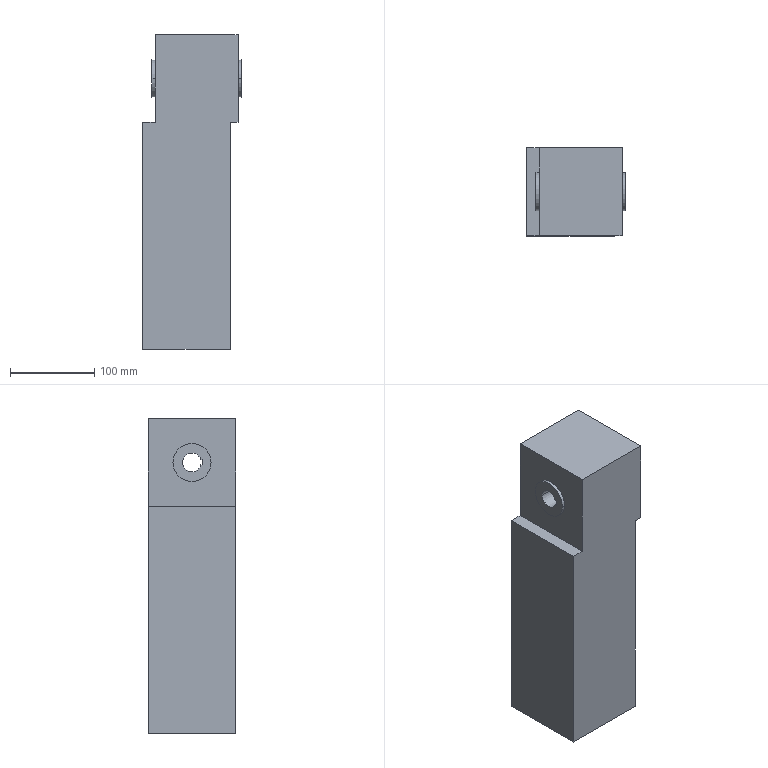Component | SolidWorks | LowerSideBeltXG-XG1-1_ServoMotor100ZJ-1 | 1 solid | 33 faces | box 117 x 104 x 373 mm | volume 3938315 mm3 | plane 19 | cylinder 14 | commonest cylinder face diameters 9 x8 45 x4 22 x2
build123d program:
from build123d import *

# Parameters (mm, degrees)
SKETCH1_W           = 104
SKETCH1_H           = 104
BOSS_EXTRUDE1_DEPTH = 373
SKETCH2_W           = 104
SKETCH2_H           = 104
BOSS_EXTRUDE2_DEPTH = 9
SKETCH3_R           = 22.5
BOSS_EXTRUDE3_DEPTH = 4
SKETCH4_W           = 15
SKETCH4_H           = 104
CUT_EXTRUDE1_DEPTH  = 104
BOSS_EXTRUDE4_START = 4
SKETCH5_R           = 22.5
BOSS_EXTRUDE4_DEPTH = 4
CUT_EXTRUDE2_DEPTH  = 395.363
SKETCH7_R           = 4.5
CUT_EXTRUDE3_DEPTH  = 10


with BuildPart() as part:
    # Sketch1 → Boss-Extrude1 (new body)
    with BuildSketch(Plane.XY):
        Rectangle(SKETCH1_W, SKETCH1_H)
    extrude(amount=BOSS_EXTRUDE1_DEPTH)

    # Sketch2 → Boss-Extrude2 (add)
    with BuildSketch(Plane.ZY.offset(52)):
        with Locations((321, 0)):
            Rectangle(SKETCH2_W, SKETCH2_H)
    extrude(amount=BOSS_EXTRUDE2_DEPTH)

    # Sketch3 → Boss-Extrude3 (add)
    with BuildSketch(Plane.ZY.offset(61)):
        with Locations(Location((321, 0, 0), (0, 0, 90))):
            Circle(SKETCH3_R)
    extrude(amount=BOSS_EXTRUDE3_DEPTH)

    # Sketch4 → Cut-Extrude1 (cut)
    with BuildSketch(Plane.XY.offset(373)):
        with Locations((44.5, 0)):
            Rectangle(SKETCH4_W, SKETCH4_H)
    extrude(amount=-CUT_EXTRUDE1_DEPTH, mode=Mode.SUBTRACT)

    # Sketch5 → Boss-Extrude4 (add)
    with BuildSketch(Plane(origin=(37, 0, 0), x_dir=(0, 0, -1), z_dir=(1, 0, 0)).offset(BOSS_EXTRUDE4_START)):
        with Locations(Location((-321, 0, 0), (0, 0, 90))):
            Circle(SKETCH5_R)
    extrude(amount=-BOSS_EXTRUDE4_DEPTH)

    # Sketch6 → Cut-Extrude2 (cut, through all)
    with BuildSketch(Plane.ZY.offset(65)):
        with BuildLine():
            Line((318, 12.5), (324, 12.5))
            Line((324, 12.5), (324, 10.583))
            ThreePointArc((324, 10.583), (321, -11), (318, 10.583))
            Line((318, 10.583), (318, 12.5))
        make_face()
    extrude(amount=-CUT_EXTRUDE2_DEPTH, mode=Mode.SUBTRACT)

    # Sketch7 → Cut-Extrude3 (cut)
    with BuildSketch(Plane.ZY.offset(61)):
        with Locations(Location((278.574, 42.426, 0), (0, 0, 270))):
            Circle(SKETCH7_R)
        with Locations(Location((363.426, 42.426, 0), (0, 0, 270))):
            Circle(SKETCH7_R)
        with Locations(Location((363.426, -42.426, 0), (0, 0, 270))):
            Circle(SKETCH7_R)
        with Locations(Location((278.574, -42.426, 0), (0, 0, 270))):
            Circle(SKETCH7_R)
    extrude(amount=-CUT_EXTRUDE3_DEPTH, mode=Mode.SUBTRACT)


solid = part.part

# Placed as in the assembly
solid = solid.moved(Location((-454.22, 625, -207), (0, 0, 180)))
STEP:
#1=COLOUR_RGB('',0.7922,0.8196,0.9333);
#2=FILL_AREA_STYLE_COLOUR('',#1);
#3=FILL_AREA_STYLE('',(#2));
#4=SURFACE_STYLE_FILL_AREA(#3);
#5=SURFACE_SIDE_STYLE('',(#4));
#6=SURFACE_STYLE_USAGE(.BOTH.,#5);
#7=PRESENTATION_STYLE_ASSIGNMENT((#6));
#8=CARTESIAN_POINT('',(-15.875,22.759,6.159));
#9=VERTEX_POINT('',#8);
#10=CARTESIAN_POINT('',(-15.875,23.113,6.159));
#11=VERTEX_POINT('',#10);
#12=CARTESIAN_POINT('',(-15.875,22.936,6.159));
#13=DIRECTION('',(1.,0.,0.));
#14=DIRECTION('',(0.,1.,0.));
#15=AXIS2_PLACEMENT_3D('',#12,#13,#14);
#16=CIRCLE('',#15,0.1772);
#17=EDGE_CURVE('',#9,#11,#16,.T.);
#18=ORIENTED_EDGE('',*,*,#17,.F.);
#19=CARTESIAN_POINT('',(-15.481,22.759,6.159));
#20=VERTEX_POINT('',#19);
#21=CARTESIAN_POINT('',(-15.875,22.759,6.159));
#22=DIRECTION('',(1.,0.,0.));
#23=VECTOR('',#22,39.37);
#24=LINE('',#21,#23);
#25=EDGE_CURVE('',#9,#20,#24,.T.);
#26=ORIENTED_EDGE('',*,*,#25,.T.);
#27=CARTESIAN_POINT('',(-15.481,23.113,6.159));
#28=VERTEX_POINT('',#27);
#29=CARTESIAN_POINT('',(-15.481,22.936,6.159));
#30=DIRECTION('',(1.,0.,0.));
#31=DIRECTION('',(0.,1.,0.));
#32=AXIS2_PLACEMENT_3D('',#29,#30,#31);
#33=CIRCLE('',#32,0.1772);
#34=EDGE_CURVE('',#20,#28,#33,.T.);
#35=ORIENTED_EDGE('',*,*,#34,.T.);
#36=CARTESIAN_POINT('',(-15.875,23.113,6.159));
#37=DIRECTION('',(1.,0.,0.));
#38=VECTOR('',#37,39.37);
#39=LINE('',#36,#38);
#40=EDGE_CURVE('',#11,#28,#39,.T.);
#41=ORIENTED_EDGE('',*,*,#40,.F.);
#42=EDGE_LOOP('',(#18,#26,#35,#41));
#43=FACE_OUTER_BOUND('',#42,.T.);
#44=CARTESIAN_POINT('',(-15.875,22.936,6.159));
#45=DIRECTION('',(1.,0.,0.));
#46=DIRECTION('',(0.,1.,0.));
#47=AXIS2_PLACEMENT_3D('',#44,#45,#46);
#48=CYLINDRICAL_SURFACE('',#47,0.1772);
#49=ADVANCED_FACE('',(#43),#48,.F.);
#50=CARTESIAN_POINT('',(-15.875,26.099,6.159));
#51=VERTEX_POINT('',#50);
#52=CARTESIAN_POINT('',(-15.875,26.454,6.159));
#53=VERTEX_POINT('',#52);
#54=CARTESIAN_POINT('',(-15.875,26.277,6.159));
#55=DIRECTION('',(1.,0.,0.));
#56=DIRECTION('',(0.,1.,0.));
#57=AXIS2_PLACEMENT_3D('',#54,#55,#56);
#58=CIRCLE('',#57,0.1772);
#59=EDGE_CURVE('',#51,#53,#58,.T.);
#60=ORIENTED_EDGE('',*,*,#59,.F.);
#61=CARTESIAN_POINT('',(-15.481,26.099,6.159));
#62=VERTEX_POINT('',#61);
#63=CARTESIAN_POINT('',(-15.875,26.099,6.159));
#64=DIRECTION('',(1.,0.,0.));
#65=VECTOR('',#64,39.37);
#66=LINE('',#63,#65);
#67=EDGE_CURVE('',#51,#62,#66,.T.);
#68=ORIENTED_EDGE('',*,*,#67,.T.);
#69=CARTESIAN_POINT('',(-15.481,26.454,6.159));
#70=VERTEX_POINT('',#69);
#71=CARTESIAN_POINT('',(-15.481,26.277,6.159));
#72=DIRECTION('',(1.,0.,0.));
#73=DIRECTION('',(0.,1.,0.));
#74=AXIS2_PLACEMENT_3D('',#71,#72,#73);
#75=CIRCLE('',#74,0.1772);
#76=EDGE_CURVE('',#62,#70,#75,.T.);
#77=ORIENTED_EDGE('',*,*,#76,.T.);
#78=CARTESIAN_POINT('',(-15.875,26.454,6.159));
#79=DIRECTION('',(1.,0.,0.));
#80=VECTOR('',#79,39.37);
#81=LINE('',#78,#80);
#82=EDGE_CURVE('',#53,#70,#81,.T.);
#83=ORIENTED_EDGE('',*,*,#82,.F.);
#84=EDGE_LOOP('',(#60,#68,#77,#83));
#85=FACE_OUTER_BOUND('',#84,.T.);
#86=CARTESIAN_POINT('',(-15.875,26.277,6.159));
#87=DIRECTION('',(1.,0.,0.));
#88=DIRECTION('',(0.,1.,0.));
#89=AXIS2_PLACEMENT_3D('',#86,#87,#88);
#90=CYLINDRICAL_SURFACE('',#89,0.1772);
#91=ADVANCED_FACE('',(#85),#90,.F.);
#92=CARTESIAN_POINT('',(-15.875,26.099,2.818));
#93=VERTEX_POINT('',#92);
#94=CARTESIAN_POINT('',(-15.875,26.454,2.818));
#95=VERTEX_POINT('',#94);
#96=CARTESIAN_POINT('',(-15.875,26.277,2.818));
#97=DIRECTION('',(1.,0.,0.));
#98=DIRECTION('',(0.,1.,0.));
#99=AXIS2_PLACEMENT_3D('',#96,#97,#98);
#100=CIRCLE('',#99,0.1772);
#101=EDGE_CURVE('',#93,#95,#100,.T.);
#102=ORIENTED_EDGE('',*,*,#101,.F.);
#103=CARTESIAN_POINT('',(-15.481,26.099,2.818));
#104=VERTEX_POINT('',#103);
#105=CARTESIAN_POINT('',(-15.875,26.099,2.818));
#106=DIRECTION('',(1.,0.,0.));
#107=VECTOR('',#106,39.37);
#108=LINE('',#105,#107);
#109=EDGE_CURVE('',#93,#104,#108,.T.);
#110=ORIENTED_EDGE('',*,*,#109,.T.);
#111=CARTESIAN_POINT('',(-15.481,26.454,2.818));
#112=VERTEX_POINT('',#111);
#113=CARTESIAN_POINT('',(-15.481,26.277,2.818));
#114=DIRECTION('',(1.,0.,0.));
#115=DIRECTION('',(0.,1.,0.));
#116=AXIS2_PLACEMENT_3D('',#113,#114,#115);
#117=CIRCLE('',#116,0.1772);
#118=EDGE_CURVE('',#104,#112,#117,.T.);
#119=ORIENTED_EDGE('',*,*,#118,.T.);
#120=CARTESIAN_POINT('',(-15.875,26.454,2.818));
#121=DIRECTION('',(1.,0.,0.));
#122=VECTOR('',#121,39.37);
#123=LINE('',#120,#122);
#124=EDGE_CURVE('',#95,#112,#123,.T.);
#125=ORIENTED_EDGE('',*,*,#124,.F.);
#126=EDGE_LOOP('',(#102,#110,#119,#125));
#127=FACE_OUTER_BOUND('',#126,.T.);
#128=CARTESIAN_POINT('',(-15.875,26.277,2.818));
#129=DIRECTION('',(1.,0.,0.));
#130=DIRECTION('',(0.,1.,0.));
#131=AXIS2_PLACEMENT_3D('',#128,#129,#130);
#132=CYLINDRICAL_SURFACE('',#131,0.1772);
#133=ADVANCED_FACE('',(#127),#132,.F.);
#134=CARTESIAN_POINT('',(-15.875,22.759,2.818));
#135=VERTEX_POINT('',#134);
#136=CARTESIAN_POINT('',(-15.875,23.113,2.818));
#137=VERTEX_POINT('',#136);
#138=CARTESIAN_POINT('',(-15.875,22.936,2.818));
#139=DIRECTION('',(1.,0.,0.));
#140=DIRECTION('',(0.,1.,0.));
#141=AXIS2_PLACEMENT_3D('',#138,#139,#140);
#142=CIRCLE('',#141,0.1772);
#143=EDGE_CURVE('',#135,#137,#142,.T.);
#144=ORIENTED_EDGE('',*,*,#143,.F.);
#145=CARTESIAN_POINT('',(-15.481,22.759,2.818));
#146=VERTEX_POINT('',#145);
#147=CARTESIAN_POINT('',(-15.875,22.759,2.818));
#148=DIRECTION('',(1.,0.,0.));
#149=VECTOR('',#148,39.37);
#150=LINE('',#147,#149);
#151=EDGE_CURVE('',#135,#146,#150,.T.);
#152=ORIENTED_EDGE('',*,*,#151,.T.);
#153=CARTESIAN_POINT('',(-15.481,23.113,2.818));
#154=VERTEX_POINT('',#153);
#155=CARTESIAN_POINT('',(-15.481,22.936,2.818));
#156=DIRECTION('',(1.,0.,0.));
#157=DIRECTION('',(0.,1.,0.));
#158=AXIS2_PLACEMENT_3D('',#155,#156,#157);
#159=CIRCLE('',#158,0.1772);
#160=EDGE_CURVE('',#146,#154,#159,.T.);
#161=ORIENTED_EDGE('',*,*,#160,.T.);
#162=CARTESIAN_POINT('',(-15.875,23.113,2.818));
#163=DIRECTION('',(1.,0.,0.));
#164=VECTOR('',#163,39.37);
#165=LINE('',#162,#164);
#166=EDGE_CURVE('',#137,#154,#165,.T.);
#167=ORIENTED_EDGE('',*,*,#166,.F.);
#168=EDGE_LOOP('',(#144,#152,#161,#167));
#169=FACE_OUTER_BOUND('',#168,.T.);
#170=CARTESIAN_POINT('',(-15.875,22.936,2.818));
#171=DIRECTION('',(1.,0.,0.));
#172=DIRECTION('',(0.,1.,0.));
#173=AXIS2_PLACEMENT_3D('',#170,#171,#172);
#174=CYLINDRICAL_SURFACE('',#173,0.1772);
#175=ADVANCED_FACE('',(#169),#174,.F.);
#176=CARTESIAN_POINT('',(-19.497,24.19,4.606));
#177=VERTEX_POINT('',#176);
#178=CARTESIAN_POINT('',(-19.497,25.039,4.488));
#179=VERTEX_POINT('',#178);
#180=CARTESIAN_POINT('',(-19.497,24.606,4.488));
#181=DIRECTION('',(-1.,-0.,-0.));
#182=DIRECTION('',(0.,-1.,0.));
#183=AXIS2_PLACEMENT_3D('',#180,#181,#182);
#184=CIRCLE('',#183,0.4331);
#185=EDGE_CURVE('',#177,#179,#184,.T.);
#186=ORIENTED_EDGE('',*,*,#185,.T.);
#187=CARTESIAN_POINT('',(-15.324,25.039,4.488));
#188=VERTEX_POINT('',#187);
#189=CARTESIAN_POINT('',(-19.93,25.039,4.488));
#190=DIRECTION('',(1.,0.,0.));
#191=VECTOR('',#190,39.37);
#192=LINE('',#189,#191);
#193=EDGE_CURVE('',#179,#188,#192,.T.);
#194=ORIENTED_EDGE('',*,*,#193,.T.);
#195=CARTESIAN_POINT('',(-15.324,24.19,4.606));
#196=VERTEX_POINT('',#195);
#197=CARTESIAN_POINT('',(-15.324,24.606,4.488));
#198=DIRECTION('',(1.,0.,0.));
#199=DIRECTION('',(0.,1.,0.));
#200=AXIS2_PLACEMENT_3D('',#197,#198,#199);
#201=CIRCLE('',#200,0.4331);
#202=EDGE_CURVE('',#188,#196,#201,.T.);
#203=ORIENTED_EDGE('',*,*,#202,.T.);
#204=CARTESIAN_POINT('',(-19.93,24.19,4.606));
#205=DIRECTION('',(1.,0.,0.));
#206=VECTOR('',#205,39.37);
#207=LINE('',#204,#206);
#208=EDGE_CURVE('',#177,#196,#207,.T.);
#209=ORIENTED_EDGE('',*,*,#208,.F.);
#210=EDGE_LOOP('',(#186,#194,#203,#209));
#211=FACE_OUTER_BOUND('',#210,.T.);
#212=CARTESIAN_POINT('',(-19.93,24.606,4.488));
#213=DIRECTION('',(1.,0.,0.));
#214=DIRECTION('',(0.,1.,0.));
#215=AXIS2_PLACEMENT_3D('',#212,#213,#214);
#216=CYLINDRICAL_SURFACE('',#215,0.4331);
#217=ADVANCED_FACE('',(#211),#216,.F.);
#218=CARTESIAN_POINT('',(-19.497,23.72,4.488));
#219=VERTEX_POINT('',#218);
#220=CARTESIAN_POINT('',(-19.497,25.492,4.488));
#221=VERTEX_POINT('',#220);
#222=CARTESIAN_POINT('',(-19.497,24.606,4.488));
#223=DIRECTION('',(-1.,-0.,-0.));
#224=DIRECTION('',(0.,-1.,0.));
#225=AXIS2_PLACEMENT_3D('',#222,#223,#224);
#226=CIRCLE('',#225,0.8858);
#227=EDGE_CURVE('',#219,#221,#226,.T.);
#228=ORIENTED_EDGE('',*,*,#227,.F.);
#229=CARTESIAN_POINT('',(-19.339,23.72,4.488));
#230=VERTEX_POINT('',#229);
#231=CARTESIAN_POINT('',(-19.497,23.72,4.488));
#232=DIRECTION('',(1.,0.,0.));
#233=VECTOR('',#232,39.37);
#234=LINE('',#231,#233);
#235=EDGE_CURVE('',#219,#230,#234,.T.);
#236=ORIENTED_EDGE('',*,*,#235,.T.);
#237=CARTESIAN_POINT('',(-19.339,25.492,4.488));
#238=VERTEX_POINT('',#237);
#239=CARTESIAN_POINT('',(-19.339,24.606,4.488));
#240=DIRECTION('',(-1.,-0.,-0.));
#241=DIRECTION('',(-0.,1.,0.));
#242=AXIS2_PLACEMENT_3D('',#239,#240,#241);
#243=CIRCLE('',#242,0.8858);
#244=EDGE_CURVE('',#230,#238,#243,.T.);
#245=ORIENTED_EDGE('',*,*,#244,.T.);
#246=CARTESIAN_POINT('',(-19.497,25.492,4.488));
#247=DIRECTION('',(1.,0.,0.));
#248=VECTOR('',#247,39.37);
#249=LINE('',#246,#248);
#250=EDGE_CURVE('',#221,#238,#249,.T.);
#251=ORIENTED_EDGE('',*,*,#250,.F.);
#252=EDGE_LOOP('',(#228,#236,#245,#251));
#253=FACE_OUTER_BOUND('',#252,.T.);
#254=CARTESIAN_POINT('',(-19.497,24.606,4.488));
#255=DIRECTION('',(1.,0.,0.));
#256=DIRECTION('',(-0.,1.,0.));
#257=AXIS2_PLACEMENT_3D('',#254,#255,#256);
#258=CYLINDRICAL_SURFACE('',#257,0.8858);
#259=ADVANCED_FACE('',(#253),#258,.T.);
#260=CARTESIAN_POINT('',(-15.324,25.492,4.488));
#261=VERTEX_POINT('',#260);
#262=CARTESIAN_POINT('',(-15.324,23.72,4.488));
#263=VERTEX_POINT('',#262);
#264=CARTESIAN_POINT('',(-15.324,24.606,4.488));
#265=DIRECTION('',(1.,0.,0.));
#266=DIRECTION('',(-0.,1.,0.));
#267=AXIS2_PLACEMENT_3D('',#264,#265,#266);
#268=CIRCLE('',#267,0.8858);
#269=EDGE_CURVE('',#261,#263,#268,.T.);
#270=ORIENTED_EDGE('',*,*,#269,.F.);
#271=CARTESIAN_POINT('',(-15.481,25.492,4.488));
#272=VERTEX_POINT('',#271);
#273=CARTESIAN_POINT('',(-15.324,25.492,4.488));
#274=DIRECTION('',(-1.,-0.,-0.));
#275=VECTOR('',#274,39.37);
#276=LINE('',#273,#275);
#277=EDGE_CURVE('',#261,#272,#276,.T.);
#278=ORIENTED_EDGE('',*,*,#277,.T.);
#279=CARTESIAN_POINT('',(-15.481,23.72,4.488));
#280=VERTEX_POINT('',#279);
#281=CARTESIAN_POINT('',(-15.481,24.606,4.488));
#282=DIRECTION('',(1.,0.,0.));
#283=DIRECTION('',(0.,-1.,0.));
#284=AXIS2_PLACEMENT_3D('',#281,#282,#283);
#285=CIRCLE('',#284,0.8858);
#286=EDGE_CURVE('',#272,#280,#285,.T.);
#287=ORIENTED_EDGE('',*,*,#286,.T.);
#288=CARTESIAN_POINT('',(-15.324,23.72,4.488));
#289=DIRECTION('',(-1.,-0.,-0.));
#290=VECTOR('',#289,39.37);
#291=LINE('',#288,#290);
#292=EDGE_CURVE('',#263,#280,#291,.T.);
#293=ORIENTED_EDGE('',*,*,#292,.F.);
#294=EDGE_LOOP('',(#270,#278,#287,#293));
#295=FACE_OUTER_BOUND('',#294,.T.);
#296=CARTESIAN_POINT('',(-15.324,24.606,4.488));
#297=DIRECTION('',(-1.,-0.,-0.));
#298=DIRECTION('',(0.,-1.,0.));
#299=AXIS2_PLACEMENT_3D('',#296,#297,#298);
#300=CYLINDRICAL_SURFACE('',#299,0.8858);
#301=ADVANCED_FACE('',(#295),#300,.T.);
#302=CARTESIAN_POINT('',(-15.835,22.559,2.441));
#303=VERTEX_POINT('',#302);
#304=CARTESIAN_POINT('',(-15.835,26.654,2.441));
#305=VERTEX_POINT('',#304);
#306=CARTESIAN_POINT('',(-15.835,22.559,2.441));
#307=DIRECTION('',(-0.,1.,0.));
#308=VECTOR('',#307,39.37);
#309=LINE('',#306,#308);
#310=EDGE_CURVE('',#303,#305,#309,.T.);
#311=ORIENTED_EDGE('',*,*,#310,.F.);
#312=CARTESIAN_POINT('',(-15.835,22.559,-8.15));
#313=VERTEX_POINT('',#312);
#314=CARTESIAN_POINT('',(-15.835,22.559,6.535));
#315=DIRECTION('',(0.,0.,-1.));
#316=VECTOR('',#315,39.37);
#317=LINE('',#314,#316);
#318=EDGE_CURVE('',#303,#313,#317,.T.);
#319=ORIENTED_EDGE('',*,*,#318,.T.);
#320=CARTESIAN_POINT('',(-15.835,26.654,-8.15));
#321=VERTEX_POINT('',#320);
#322=CARTESIAN_POINT('',(-15.835,22.559,-8.15));
#323=DIRECTION('',(-0.,1.,0.));
#324=VECTOR('',#323,39.37);
#325=LINE('',#322,#324);
#326=EDGE_CURVE('',#313,#321,#325,.T.);
#327=ORIENTED_EDGE('',*,*,#326,.T.);
#328=CARTESIAN_POINT('',(-15.835,26.654,6.535));
#329=DIRECTION('',(0.,0.,-1.));
#330=VECTOR('',#329,39.37);
#331=LINE('',#328,#330);
#332=EDGE_CURVE('',#305,#321,#331,.T.);
#333=ORIENTED_EDGE('',*,*,#332,.F.);
#334=EDGE_LOOP('',(#311,#319,#327,#333));
#335=FACE_OUTER_BOUND('',#334,.T.);
#336=CARTESIAN_POINT('',(-15.835,22.559,6.535));
#337=DIRECTION('',(-1.,-0.,-0.));
#338=DIRECTION('',(0.,-1.,-0.));
#339=AXIS2_PLACEMENT_3D('',#336,#337,#338);
#340=PLANE('',#339);
#341=ADVANCED_FACE('',(#335),#340,.F.);
#342=CARTESIAN_POINT('',(-19.93,22.559,2.441));
#343=VERTEX_POINT('',#342);
#344=CARTESIAN_POINT('',(-19.93,22.559,-8.15));
#345=VERTEX_POINT('',#344);
#346=CARTESIAN_POINT('',(-19.93,22.559,6.535));
#347=DIRECTION('',(0.,0.,-1.));
#348=VECTOR('',#347,39.37);
#349=LINE('',#346,#348);
#350=EDGE_CURVE('',#343,#345,#349,.T.);
#351=ORIENTED_EDGE('',*,*,#350,.F.);
#352=CARTESIAN_POINT('',(-19.93,26.654,2.441));
#353=VERTEX_POINT('',#352);
#354=CARTESIAN_POINT('',(-19.93,22.559,2.441));
#355=DIRECTION('',(0.,-1.,-0.));
#356=VECTOR('',#355,39.37);
#357=LINE('',#354,#356);
#358=EDGE_CURVE('',#353,#343,#357,.T.);
#359=ORIENTED_EDGE('',*,*,#358,.F.);
#360=CARTESIAN_POINT('',(-19.93,26.654,-8.15));
#361=VERTEX_POINT('',#360);
#362=CARTESIAN_POINT('',(-19.93,26.654,6.535));
#363=DIRECTION('',(0.,0.,-1.));
#364=VECTOR('',#363,39.37);
#365=LINE('',#362,#364);
#366=EDGE_CURVE('',#353,#361,#365,.T.);
#367=ORIENTED_EDGE('',*,*,#366,.T.);
#368=CARTESIAN_POINT('',(-19.93,22.559,-8.15));
#369=DIRECTION('',(0.,-1.,-0.));
#370=VECTOR('',#369,39.37);
#371=LINE('',#368,#370);
#372=EDGE_CURVE('',#361,#345,#371,.T.);
#373=ORIENTED_EDGE('',*,*,#372,.T.);
#374=EDGE_LOOP('',(#351,#359,#367,#373));
#375=FACE_OUTER_BOUND('',#374,.T.);
#376=CARTESIAN_POINT('',(-19.93,22.559,6.535));
#377=DIRECTION('',(1.,0.,0.));
#378=DIRECTION('',(-0.,1.,0.));
#379=AXIS2_PLACEMENT_3D('',#376,#377,#378);
#380=PLANE('',#379);
#381=ADVANCED_FACE('',(#375),#380,.F.);
#382=CARTESIAN_POINT('',(-19.339,22.559,6.535));
#383=VERTEX_POINT('',#382);
#384=CARTESIAN_POINT('',(-15.481,22.559,6.535));
#385=VERTEX_POINT('',#384);
#386=CARTESIAN_POINT('',(-15.835,22.559,6.535));
#387=DIRECTION('',(1.,0.,0.));
#388=VECTOR('',#387,39.37);
#389=LINE('',#386,#388);
#390=EDGE_CURVE('',#383,#385,#389,.T.);
#391=ORIENTED_EDGE('',*,*,#390,.F.);
#392=CARTESIAN_POINT('',(-19.339,22.559,2.441));
#393=VERTEX_POINT('',#392);
#394=CARTESIAN_POINT('',(-19.339,22.559,2.441));
#395=DIRECTION('',(-0.,-0.,1.));
#396=VECTOR('',#395,39.37);
#397=LINE('',#394,#396);
#398=EDGE_CURVE('',#393,#383,#397,.T.);
#399=ORIENTED_EDGE('',*,*,#398,.F.);
#400=CARTESIAN_POINT('',(-19.93,22.559,2.441));
#401=DIRECTION('',(1.,0.,0.));
#402=VECTOR('',#401,39.37);
#403=LINE('',#400,#402);
#404=EDGE_CURVE('',#343,#393,#403,.T.);
#405=ORIENTED_EDGE('',*,*,#404,.F.);
#406=ORIENTED_EDGE('',*,*,#350,.T.);
#407=CARTESIAN_POINT('',(-15.835,22.559,-8.15));
#408=DIRECTION('',(1.,0.,0.));
#409=VECTOR('',#408,39.37);
#410=LINE('',#407,#409);
#411=EDGE_CURVE('',#345,#313,#410,.T.);
#412=ORIENTED_EDGE('',*,*,#411,.T.);
#413=ORIENTED_EDGE('',*,*,#318,.F.);
#414=CARTESIAN_POINT('',(-15.481,22.559,2.441));
#415=VERTEX_POINT('',#414);
#416=CARTESIAN_POINT('',(-15.481,22.559,2.441));
#417=DIRECTION('',(-1.,-0.,-0.));
#418=VECTOR('',#417,39.37);
#419=LINE('',#416,#418);
#420=EDGE_CURVE('',#415,#303,#419,.T.);
#421=ORIENTED_EDGE('',*,*,#420,.F.);
#422=CARTESIAN_POINT('',(-15.481,22.559,6.535));
#423=DIRECTION('',(0.,0.,-1.));
#424=VECTOR('',#423,39.37);
#425=LINE('',#422,#424);
#426=EDGE_CURVE('',#385,#415,#425,.T.);
#427=ORIENTED_EDGE('',*,*,#426,.F.);
#428=EDGE_LOOP('',(#391,#399,#405,#406,#412,#413,#421,#427));
#429=FACE_OUTER_BOUND('',#428,.T.);
#430=CARTESIAN_POINT('',(-15.835,22.559,6.535));
#431=DIRECTION('',(-0.,1.,0.));
#432=DIRECTION('',(0.,0.,-1.));
#433=AXIS2_PLACEMENT_3D('',#430,#431,#432);
#434=PLANE('',#433);
#435=ADVANCED_FACE('',(#429),#434,.F.);
#436=CARTESIAN_POINT('',(-19.339,26.654,2.441));
#437=VERTEX_POINT('',#436);
#438=CARTESIAN_POINT('',(-19.93,26.654,2.441));
#439=DIRECTION('',(-1.,-0.,-0.));
#440=VECTOR('',#439,39.37);
#441=LINE('',#438,#440);
#442=EDGE_CURVE('',#437,#353,#441,.T.);
#443=ORIENTED_EDGE('',*,*,#442,.F.);
#444=CARTESIAN_POINT('',(-19.339,26.654,6.535));
#445=VERTEX_POINT('',#444);
#446=CARTESIAN_POINT('',(-19.339,26.654,2.441));
#447=DIRECTION('',(-0.,-0.,1.));
#448=VECTOR('',#447,39.37);
#449=LINE('',#446,#448);
#450=EDGE_CURVE('',#437,#445,#449,.T.);
#451=ORIENTED_EDGE('',*,*,#450,.T.);
#452=CARTESIAN_POINT('',(-15.481,26.654,6.535));
#453=VERTEX_POINT('',#452);
#454=CARTESIAN_POINT('',(-15.835,26.654,6.535));
#455=DIRECTION('',(-1.,-0.,-0.));
#456=VECTOR('',#455,39.37);
#457=LINE('',#454,#456);
#458=EDGE_CURVE('',#453,#445,#457,.T.);
#459=ORIENTED_EDGE('',*,*,#458,.F.);
#460=CARTESIAN_POINT('',(-15.481,26.654,2.441));
#461=VERTEX_POINT('',#460);
#462=CARTESIAN_POINT('',(-15.481,26.654,6.535));
#463=DIRECTION('',(-0.,-0.,1.));
#464=VECTOR('',#463,39.37);
#465=LINE('',#462,#464);
#466=EDGE_CURVE('',#461,#453,#465,.T.);
#467=ORIENTED_EDGE('',*,*,#466,.F.);
#468=CARTESIAN_POINT('',(-15.481,26.654,2.441));
#469=DIRECTION('',(-1.,-0.,-0.));
#470=VECTOR('',#469,39.37);
#471=LINE('',#468,#470);
#472=EDGE_CURVE('',#461,#305,#471,.T.);
#473=ORIENTED_EDGE('',*,*,#472,.T.);
#474=ORIENTED_EDGE('',*,*,#332,.T.);
#475=CARTESIAN_POINT('',(-15.835,26.654,-8.15));
#476=DIRECTION('',(-1.,-0.,-0.));
#477=VECTOR('',#476,39.37);
#478=LINE('',#475,#477);
#479=EDGE_CURVE('',#321,#361,#478,.T.);
#480=ORIENTED_EDGE('',*,*,#479,.T.);
#481=ORIENTED_EDGE('',*,*,#366,.F.);
#482=EDGE_LOOP('',(#443,#451,#459,#467,#473,#474,#480,#481));
#483=FACE_OUTER_BOUND('',#482,.T.);
#484=CARTESIAN_POINT('',(-15.835,26.654,6.535));
#485=DIRECTION('',(0.,-1.,-0.));
#486=DIRECTION('',(-0.,-0.,1.));
#487=AXIS2_PLACEMENT_3D('',#484,#485,#486);
#488=PLANE('',#487);
#489=ADVANCED_FACE('',(#483),#488,.F.);
#490=CARTESIAN_POINT('',(-19.339,22.559,6.535));
#491=DIRECTION('',(-0.,1.,0.));
#492=VECTOR('',#491,39.37);
#493=LINE('',#490,#492);
#494=EDGE_CURVE('',#383,#445,#493,.T.);
#495=ORIENTED_EDGE('',*,*,#494,.F.);
#496=ORIENTED_EDGE('',*,*,#390,.T.);
#497=CARTESIAN_POINT('',(-15.481,22.559,6.535));
#498=DIRECTION('',(0.,-1.,-0.));
#499=VECTOR('',#498,39.37);
#500=LINE('',#497,#499);
#501=EDGE_CURVE('',#453,#385,#500,.T.);
#502=ORIENTED_EDGE('',*,*,#501,.F.);
#503=ORIENTED_EDGE('',*,*,#458,.T.);
#504=EDGE_LOOP('',(#495,#496,#502,#503));
#505=FACE_OUTER_BOUND('',#504,.T.);
#506=CARTESIAN_POINT('',(-17.883,24.606,6.535));
#507=DIRECTION('',(-0.,-0.,1.));
#508=DIRECTION('',(-1.,-0.,-0.));
#509=AXIS2_PLACEMENT_3D('',#506,#507,#508);
#510=PLANE('',#509);
#511=ADVANCED_FACE('',(#505),#510,.T.);
#512=ORIENTED_EDGE('',*,*,#372,.F.);
#513=ORIENTED_EDGE('',*,*,#479,.F.);
#514=ORIENTED_EDGE('',*,*,#326,.F.);
#515=ORIENTED_EDGE('',*,*,#411,.F.);
#516=EDGE_LOOP('',(#512,#513,#514,#515));
#517=FACE_OUTER_BOUND('',#516,.T.);
#518=CARTESIAN_POINT('',(-17.883,24.606,-8.15));
#519=DIRECTION('',(-0.,-0.,1.));
#520=DIRECTION('',(-1.,-0.,-0.));
#521=AXIS2_PLACEMENT_3D('',#518,#519,#520);
#522=PLANE('',#521);
#523=ADVANCED_FACE('',(#517),#522,.F.);
#524=ORIENTED_EDGE('',*,*,#310,.T.);
#525=ORIENTED_EDGE('',*,*,#472,.F.);
#526=CARTESIAN_POINT('',(-15.481,22.559,2.441));
#527=DIRECTION('',(-0.,1.,0.));
#528=VECTOR('',#527,39.37);
#529=LINE('',#526,#528);
#530=EDGE_CURVE('',#415,#461,#529,.T.);
#531=ORIENTED_EDGE('',*,*,#530,.F.);
#532=ORIENTED_EDGE('',*,*,#420,.T.);
#533=EDGE_LOOP('',(#524,#525,#531,#532));
#534=FACE_OUTER_BOUND('',#533,.T.);
#535=CARTESIAN_POINT('',(-15.481,22.559,2.441));
#536=DIRECTION('',(-0.,-0.,1.));
#537=DIRECTION('',(-1.,-0.,-0.));
#538=AXIS2_PLACEMENT_3D('',#535,#536,#537);
#539=PLANE('',#538);
#540=ADVANCED_FACE('',(#534),#539,.F.);
#541=CARTESIAN_POINT('',(-15.481,22.936,6.159));
#542=DIRECTION('',(1.,0.,0.));
#543=DIRECTION('',(0.,1.,0.));
#544=AXIS2_PLACEMENT_3D('',#541,#542,#543);
#545=CIRCLE('',#544,0.1772);
#546=EDGE_CURVE('',#28,#20,#545,.T.);
#547=ORIENTED_EDGE('',*,*,#546,.F.);
#548=ORIENTED_EDGE('',*,*,#34,.F.);
#549=EDGE_LOOP('',(#547,#548));
#550=FACE_BOUND('',#549,.T.);
#551=CARTESIAN_POINT('',(-15.481,26.277,6.159));
#552=DIRECTION('',(1.,0.,0.));
#553=DIRECTION('',(0.,1.,0.));
#554=AXIS2_PLACEMENT_3D('',#551,#552,#553);
#555=CIRCLE('',#554,0.1772);
#556=EDGE_CURVE('',#70,#62,#555,.T.);
#557=ORIENTED_EDGE('',*,*,#556,.F.);
#558=ORIENTED_EDGE('',*,*,#76,.F.);
#559=EDGE_LOOP('',(#557,#558));
#560=FACE_BOUND('',#559,.T.);
#561=CARTESIAN_POINT('',(-15.481,26.277,2.818));
#562=DIRECTION('',(1.,0.,0.));
#563=DIRECTION('',(0.,1.,0.));
#564=AXIS2_PLACEMENT_3D('',#561,#562,#563);
#565=CIRCLE('',#564,0.1772);
#566=EDGE_CURVE('',#112,#104,#565,.T.);
#567=ORIENTED_EDGE('',*,*,#566,.F.);
#568=ORIENTED_EDGE('',*,*,#118,.F.);
#569=EDGE_LOOP('',(#567,#568));
#570=FACE_BOUND('',#569,.T.);
#571=CARTESIAN_POINT('',(-15.481,22.936,2.818));
#572=DIRECTION('',(1.,0.,0.));
#573=DIRECTION('',(0.,1.,0.));
#574=AXIS2_PLACEMENT_3D('',#571,#572,#573);
#575=CIRCLE('',#574,0.1772);
#576=EDGE_CURVE('',#154,#146,#575,.T.);
#577=ORIENTED_EDGE('',*,*,#576,.F.);
#578=ORIENTED_EDGE('',*,*,#160,.F.);
#579=EDGE_LOOP('',(#577,#578));
#580=FACE_BOUND('',#579,.T.);
#581=CARTESIAN_POINT('',(-15.481,24.606,4.488));
#582=DIRECTION('',(1.,0.,0.));
#583=DIRECTION('',(0.,-1.,0.));
#584=AXIS2_PLACEMENT_3D('',#581,#582,#583);
#585=CIRCLE('',#584,0.8858);
#586=EDGE_CURVE('',#280,#272,#585,.T.);
#587=ORIENTED_EDGE('',*,*,#586,.F.);
#588=ORIENTED_EDGE('',*,*,#286,.F.);
#589=EDGE_LOOP('',(#587,#588));
#590=FACE_BOUND('',#589,.T.);
#591=ORIENTED_EDGE('',*,*,#501,.T.);
#592=ORIENTED_EDGE('',*,*,#426,.T.);
#593=ORIENTED_EDGE('',*,*,#530,.T.);
#594=ORIENTED_EDGE('',*,*,#466,.T.);
#595=EDGE_LOOP('',(#591,#592,#593,#594));
#596=FACE_OUTER_BOUND('',#595,.T.);
#597=CARTESIAN_POINT('',(-15.481,24.606,-8.15));
#598=DIRECTION('',(-1.,-0.,-0.));
#599=DIRECTION('',(0.,-1.,-0.));
#600=AXIS2_PLACEMENT_3D('',#597,#598,#599);
#601=PLANE('',#600);
#602=ADVANCED_FACE('',(#550,#560,#570,#580,#590,#596),#601,.F.);
#603=ORIENTED_EDGE('',*,*,#277,.F.);
#604=CARTESIAN_POINT('',(-15.324,24.606,4.488));
#605=DIRECTION('',(1.,0.,0.));
#606=DIRECTION('',(-0.,1.,0.));
#607=AXIS2_PLACEMENT_3D('',#604,#605,#606);
#608=CIRCLE('',#607,0.8858);
#609=EDGE_CURVE('',#263,#261,#608,.T.);
#610=ORIENTED_EDGE('',*,*,#609,.F.);
#611=ORIENTED_EDGE('',*,*,#292,.T.);
#612=ORIENTED_EDGE('',*,*,#586,.T.);
#613=EDGE_LOOP('',(#603,#610,#611,#612));
#614=FACE_OUTER_BOUND('',#613,.T.);
#615=CARTESIAN_POINT('',(-15.324,24.606,4.488));
#616=DIRECTION('',(-1.,-0.,-0.));
#617=DIRECTION('',(0.,-1.,0.));
#618=AXIS2_PLACEMENT_3D('',#615,#616,#617);
#619=CYLINDRICAL_SURFACE('',#618,0.8858);
#620=ADVANCED_FACE('',(#614),#619,.T.);
#621=CARTESIAN_POINT('',(-15.324,24.19,4.37));
#622=VERTEX_POINT('',#621);
#623=CARTESIAN_POINT('',(-15.324,24.606,4.488));
#624=DIRECTION('',(1.,0.,0.));
#625=DIRECTION('',(0.,1.,0.));
#626=AXIS2_PLACEMENT_3D('',#623,#624,#625);
#627=CIRCLE('',#626,0.4331);
#628=EDGE_CURVE('',#622,#188,#627,.T.);
#629=ORIENTED_EDGE('',*,*,#628,.F.);
#630=CARTESIAN_POINT('',(-15.324,24.114,4.37));
#631=VERTEX_POINT('',#630);
#632=CARTESIAN_POINT('',(-15.324,24.114,4.37));
#633=DIRECTION('',(-0.,1.,0.));
#634=VECTOR('',#633,39.37);
#635=LINE('',#632,#634);
#636=EDGE_CURVE('',#631,#622,#635,.T.);
#637=ORIENTED_EDGE('',*,*,#636,.F.);
#638=CARTESIAN_POINT('',(-15.324,24.114,4.606));
#639=VERTEX_POINT('',#638);
#640=CARTESIAN_POINT('',(-15.324,24.114,4.37));
#641=DIRECTION('',(0.,0.,-1.));
#642=VECTOR('',#641,39.37);
#643=LINE('',#640,#642);
#644=EDGE_CURVE('',#639,#631,#643,.T.);
#645=ORIENTED_EDGE('',*,*,#644,.F.);
#646=CARTESIAN_POINT('',(-15.324,24.114,4.606));
#647=DIRECTION('',(0.,-1.,-0.));
#648=VECTOR('',#647,39.37);
#649=LINE('',#646,#648);
#650=EDGE_CURVE('',#196,#639,#649,.T.);
#651=ORIENTED_EDGE('',*,*,#650,.F.);
#652=ORIENTED_EDGE('',*,*,#202,.F.);
#653=EDGE_LOOP('',(#629,#637,#645,#651,#652));
#654=FACE_BOUND('',#653,.T.);
#655=ORIENTED_EDGE('',*,*,#609,.T.);
#656=ORIENTED_EDGE('',*,*,#269,.T.);
#657=EDGE_LOOP('',(#655,#656));
#658=FACE_OUTER_BOUND('',#657,.T.);
#659=CARTESIAN_POINT('',(-15.324,24.606,4.488));
#660=DIRECTION('',(1.,0.,0.));
#661=DIRECTION('',(-0.,1.,0.));
#662=AXIS2_PLACEMENT_3D('',#659,#660,#661);
#663=PLANE('',#662);
#664=ADVANCED_FACE('',(#654,#658),#663,.T.);
#665=CARTESIAN_POINT('',(-19.339,24.606,4.488));
#666=DIRECTION('',(-1.,-0.,-0.));
#667=DIRECTION('',(-0.,1.,0.));
#668=AXIS2_PLACEMENT_3D('',#665,#666,#667);
#669=CIRCLE('',#668,0.8858);
#670=EDGE_CURVE('',#238,#230,#669,.T.);
#671=ORIENTED_EDGE('',*,*,#670,.F.);
#672=ORIENTED_EDGE('',*,*,#244,.F.);
#673=EDGE_LOOP('',(#671,#672));
#674=FACE_BOUND('',#673,.T.);
#675=ORIENTED_EDGE('',*,*,#494,.T.);
#676=ORIENTED_EDGE('',*,*,#450,.F.);
#677=CARTESIAN_POINT('',(-19.339,22.559,2.441));
#678=DIRECTION('',(-0.,1.,0.));
#679=VECTOR('',#678,39.37);
#680=LINE('',#677,#679);
#681=EDGE_CURVE('',#393,#437,#680,.T.);
#682=ORIENTED_EDGE('',*,*,#681,.F.);
#683=ORIENTED_EDGE('',*,*,#398,.T.);
#684=EDGE_LOOP('',(#675,#676,#682,#683));
#685=FACE_OUTER_BOUND('',#684,.T.);
#686=CARTESIAN_POINT('',(-19.339,22.559,2.441));
#687=DIRECTION('',(1.,0.,0.));
#688=DIRECTION('',(-0.,1.,0.));
#689=AXIS2_PLACEMENT_3D('',#686,#687,#688);
#690=PLANE('',#689);
#691=ADVANCED_FACE('',(#674,#685),#690,.F.);
#692=ORIENTED_EDGE('',*,*,#358,.T.);
#693=ORIENTED_EDGE('',*,*,#404,.T.);
#694=ORIENTED_EDGE('',*,*,#681,.T.);
#695=ORIENTED_EDGE('',*,*,#442,.T.);
#696=EDGE_LOOP('',(#692,#693,#694,#695));
#697=FACE_OUTER_BOUND('',#696,.T.);
#698=CARTESIAN_POINT('',(-17.883,24.606,2.441));
#699=DIRECTION('',(0.,0.,-1.));
#700=DIRECTION('',(1.,0.,0.));
#701=AXIS2_PLACEMENT_3D('',#698,#699,#700);
#702=PLANE('',#701);
#703=ADVANCED_FACE('',(#697),#702,.F.);
#704=ORIENTED_EDGE('',*,*,#235,.F.);
#705=CARTESIAN_POINT('',(-19.497,24.606,4.488));
#706=DIRECTION('',(-1.,-0.,-0.));
#707=DIRECTION('',(0.,-1.,0.));
#708=AXIS2_PLACEMENT_3D('',#705,#706,#707);
#709=CIRCLE('',#708,0.8858);
#710=EDGE_CURVE('',#221,#219,#709,.T.);
#711=ORIENTED_EDGE('',*,*,#710,.F.);
#712=ORIENTED_EDGE('',*,*,#250,.T.);
#713=ORIENTED_EDGE('',*,*,#670,.T.);
#714=EDGE_LOOP('',(#704,#711,#712,#713));
#715=FACE_OUTER_BOUND('',#714,.T.);
#716=CARTESIAN_POINT('',(-19.497,24.606,4.488));
#717=DIRECTION('',(1.,0.,0.));
#718=DIRECTION('',(-0.,1.,0.));
#719=AXIS2_PLACEMENT_3D('',#716,#717,#718);
#720=CYLINDRICAL_SURFACE('',#719,0.8858);
#721=ADVANCED_FACE('',(#715),#720,.T.);
#722=ORIENTED_EDGE('',*,*,#185,.F.);
#723=CARTESIAN_POINT('',(-19.497,24.114,4.606));
#724=VERTEX_POINT('',#723);
#725=CARTESIAN_POINT('',(-19.497,24.606,4.606));
#726=DIRECTION('',(-0.,1.,0.));
#727=VECTOR('',#726,39.37);
#728=LINE('',#725,#727);
#729=EDGE_CURVE('',#724,#177,#728,.T.);
#730=ORIENTED_EDGE('',*,*,#729,.F.);
#731=CARTESIAN_POINT('',(-19.497,24.114,4.37));
#732=VERTEX_POINT('',#731);
#733=CARTESIAN_POINT('',(-19.497,24.114,4.488));
#734=DIRECTION('',(-0.,-0.,1.));
#735=VECTOR('',#734,39.37);
#736=LINE('',#733,#735);
#737=EDGE_CURVE('',#732,#724,#736,.T.);
#738=ORIENTED_EDGE('',*,*,#737,.F.);
#739=CARTESIAN_POINT('',(-19.497,24.19,4.37));
#740=VERTEX_POINT('',#739);
#741=CARTESIAN_POINT('',(-19.497,24.606,4.37));
#742=DIRECTION('',(0.,-1.,-0.));
#743=VECTOR('',#742,39.37);
#744=LINE('',#741,#743);
#745=EDGE_CURVE('',#740,#732,#744,.T.);
#746=ORIENTED_EDGE('',*,*,#745,.F.);
#747=CARTESIAN_POINT('',(-19.497,24.606,4.488));
#748=DIRECTION('',(-1.,-0.,-0.));
#749=DIRECTION('',(0.,-1.,0.));
#750=AXIS2_PLACEMENT_3D('',#747,#748,#749);
#751=CIRCLE('',#750,0.4331);
#752=EDGE_CURVE('',#179,#740,#751,.T.);
#753=ORIENTED_EDGE('',*,*,#752,.F.);
#754=EDGE_LOOP('',(#722,#730,#738,#746,#753));
#755=FACE_BOUND('',#754,.T.);
#756=ORIENTED_EDGE('',*,*,#710,.T.);
#757=ORIENTED_EDGE('',*,*,#227,.T.);
#758=EDGE_LOOP('',(#756,#757));
#759=FACE_OUTER_BOUND('',#758,.T.);
#760=CARTESIAN_POINT('',(-19.497,24.606,4.488));
#761=DIRECTION('',(-1.,-0.,-0.));
#762=DIRECTION('',(0.,-1.,-0.));
#763=AXIS2_PLACEMENT_3D('',#760,#761,#762);
#764=PLANE('',#763);
#765=ADVANCED_FACE('',(#755,#759),#764,.T.);
#766=ORIENTED_EDGE('',*,*,#193,.F.);
#767=ORIENTED_EDGE('',*,*,#752,.T.);
#768=CARTESIAN_POINT('',(-19.93,24.19,4.37));
#769=DIRECTION('',(1.,0.,0.));
#770=VECTOR('',#769,39.37);
#771=LINE('',#768,#770);
#772=EDGE_CURVE('',#740,#622,#771,.T.);
#773=ORIENTED_EDGE('',*,*,#772,.T.);
#774=ORIENTED_EDGE('',*,*,#628,.T.);
#775=EDGE_LOOP('',(#766,#767,#773,#774));
#776=FACE_OUTER_BOUND('',#775,.T.);
#777=CARTESIAN_POINT('',(-19.93,24.606,4.488));
#778=DIRECTION('',(1.,0.,0.));
#779=DIRECTION('',(0.,1.,0.));
#780=AXIS2_PLACEMENT_3D('',#777,#778,#779);
#781=CYLINDRICAL_SURFACE('',#780,0.4331);
#782=ADVANCED_FACE('',(#776),#781,.F.);
#783=ORIENTED_EDGE('',*,*,#745,.T.);
#784=CARTESIAN_POINT('',(-19.93,24.114,4.37));
#785=DIRECTION('',(1.,0.,0.));
#786=VECTOR('',#785,39.37);
#787=LINE('',#784,#786);
#788=EDGE_CURVE('',#732,#631,#787,.T.);
#789=ORIENTED_EDGE('',*,*,#788,.T.);
#790=ORIENTED_EDGE('',*,*,#636,.T.);
#791=ORIENTED_EDGE('',*,*,#772,.F.);
#792=EDGE_LOOP('',(#783,#789,#790,#791));
#793=FACE_OUTER_BOUND('',#792,.T.);
#794=CARTESIAN_POINT('',(-19.93,24.114,4.37));
#795=DIRECTION('',(0.,0.,-1.));
#796=DIRECTION('',(1.,0.,0.));
#797=AXIS2_PLACEMENT_3D('',#794,#795,#796);
#798=PLANE('',#797);
#799=ADVANCED_FACE('',(#793),#798,.F.);
#800=ORIENTED_EDGE('',*,*,#737,.T.);
#801=CARTESIAN_POINT('',(-19.93,24.114,4.606));
#802=DIRECTION('',(1.,0.,0.));
#803=VECTOR('',#802,39.37);
#804=LINE('',#801,#803);
#805=EDGE_CURVE('',#724,#639,#804,.T.);
#806=ORIENTED_EDGE('',*,*,#805,.T.);
#807=ORIENTED_EDGE('',*,*,#644,.T.);
#808=ORIENTED_EDGE('',*,*,#788,.F.);
#809=EDGE_LOOP('',(#800,#806,#807,#808));
#810=FACE_OUTER_BOUND('',#809,.T.);
#811=CARTESIAN_POINT('',(-19.93,24.114,4.37));
#812=DIRECTION('',(0.,-1.,-0.));
#813=DIRECTION('',(1.,0.,0.));
#814=AXIS2_PLACEMENT_3D('',#811,#812,#813);
#815=PLANE('',#814);
#816=ADVANCED_FACE('',(#810),#815,.F.);
#817=ORIENTED_EDGE('',*,*,#729,.T.);
#818=ORIENTED_EDGE('',*,*,#208,.T.);
#819=ORIENTED_EDGE('',*,*,#650,.T.);
#820=ORIENTED_EDGE('',*,*,#805,.F.);
#821=EDGE_LOOP('',(#817,#818,#819,#820));
#822=FACE_OUTER_BOUND('',#821,.T.);
#823=CARTESIAN_POINT('',(-19.93,24.114,4.606));
#824=DIRECTION('',(-0.,-0.,1.));
#825=DIRECTION('',(-1.,-0.,-0.));
#826=AXIS2_PLACEMENT_3D('',#823,#824,#825);
#827=PLANE('',#826);
#828=ADVANCED_FACE('',(#822),#827,.F.);
#829=ORIENTED_EDGE('',*,*,#151,.F.);
#830=CARTESIAN_POINT('',(-15.875,22.936,2.818));
#831=DIRECTION('',(1.,0.,0.));
#832=DIRECTION('',(0.,1.,0.));
#833=AXIS2_PLACEMENT_3D('',#830,#831,#832);
#834=CIRCLE('',#833,0.1772);
#835=EDGE_CURVE('',#137,#135,#834,.T.);
#836=ORIENTED_EDGE('',*,*,#835,.F.);
#837=ORIENTED_EDGE('',*,*,#166,.T.);
#838=ORIENTED_EDGE('',*,*,#576,.T.);
#839=EDGE_LOOP('',(#829,#836,#837,#838));
#840=FACE_OUTER_BOUND('',#839,.T.);
#841=CARTESIAN_POINT('',(-15.875,22.936,2.818));
#842=DIRECTION('',(1.,0.,0.));
#843=DIRECTION('',(0.,1.,0.));
#844=AXIS2_PLACEMENT_3D('',#841,#842,#843);
#845=CYLINDRICAL_SURFACE('',#844,0.1772);
#846=ADVANCED_FACE('',(#840),#845,.F.);
#847=ORIENTED_EDGE('',*,*,#835,.T.);
#848=ORIENTED_EDGE('',*,*,#143,.T.);
#849=EDGE_LOOP('',(#847,#848));
#850=FACE_OUTER_BOUND('',#849,.T.);
#851=CARTESIAN_POINT('',(-15.875,22.936,2.818));
#852=DIRECTION('',(1.,0.,0.));
#853=DIRECTION('',(-0.,1.,0.));
#854=AXIS2_PLACEMENT_3D('',#851,#852,#853);
#855=PLANE('',#854);
#856=ADVANCED_FACE('',(#850),#855,.T.);
#857=ORIENTED_EDGE('',*,*,#109,.F.);
#858=CARTESIAN_POINT('',(-15.875,26.277,2.818));
#859=DIRECTION('',(1.,0.,0.));
#860=DIRECTION('',(0.,1.,0.));
#861=AXIS2_PLACEMENT_3D('',#858,#859,#860);
#862=CIRCLE('',#861,0.1772);
#863=EDGE_CURVE('',#95,#93,#862,.T.);
#864=ORIENTED_EDGE('',*,*,#863,.F.);
#865=ORIENTED_EDGE('',*,*,#124,.T.);
#866=ORIENTED_EDGE('',*,*,#566,.T.);
#867=EDGE_LOOP('',(#857,#864,#865,#866));
#868=FACE_OUTER_BOUND('',#867,.T.);
#869=CARTESIAN_POINT('',(-15.875,26.277,2.818));
#870=DIRECTION('',(1.,0.,0.));
#871=DIRECTION('',(0.,1.,0.));
#872=AXIS2_PLACEMENT_3D('',#869,#870,#871);
#873=CYLINDRICAL_SURFACE('',#872,0.1772);
#874=ADVANCED_FACE('',(#868),#873,.F.);
#875=ORIENTED_EDGE('',*,*,#863,.T.);
#876=ORIENTED_EDGE('',*,*,#101,.T.);
#877=EDGE_LOOP('',(#875,#876));
#878=FACE_OUTER_BOUND('',#877,.T.);
#879=CARTESIAN_POINT('',(-15.875,26.277,2.818));
#880=DIRECTION('',(1.,0.,0.));
#881=DIRECTION('',(-0.,1.,0.));
#882=AXIS2_PLACEMENT_3D('',#879,#880,#881);
#883=PLANE('',#882);
#884=ADVANCED_FACE('',(#878),#883,.T.);
#885=ORIENTED_EDGE('',*,*,#67,.F.);
#886=CARTESIAN_POINT('',(-15.875,26.277,6.159));
#887=DIRECTION('',(1.,0.,0.));
#888=DIRECTION('',(0.,1.,0.));
#889=AXIS2_PLACEMENT_3D('',#886,#887,#888);
#890=CIRCLE('',#889,0.1772);
#891=EDGE_CURVE('',#53,#51,#890,.T.);
#892=ORIENTED_EDGE('',*,*,#891,.F.);
#893=ORIENTED_EDGE('',*,*,#82,.T.);
#894=ORIENTED_EDGE('',*,*,#556,.T.);
#895=EDGE_LOOP('',(#885,#892,#893,#894));
#896=FACE_OUTER_BOUND('',#895,.T.);
#897=CARTESIAN_POINT('',(-15.875,26.277,6.159));
#898=DIRECTION('',(1.,0.,0.));
#899=DIRECTION('',(0.,1.,0.));
#900=AXIS2_PLACEMENT_3D('',#897,#898,#899);
#901=CYLINDRICAL_SURFACE('',#900,0.1772);
#902=ADVANCED_FACE('',(#896),#901,.F.);
#903=ORIENTED_EDGE('',*,*,#891,.T.);
#904=ORIENTED_EDGE('',*,*,#59,.T.);
#905=EDGE_LOOP('',(#903,#904));
#906=FACE_OUTER_BOUND('',#905,.T.);
#907=CARTESIAN_POINT('',(-15.875,26.277,6.159));
#908=DIRECTION('',(1.,0.,0.));
#909=DIRECTION('',(-0.,1.,0.));
#910=AXIS2_PLACEMENT_3D('',#907,#908,#909);
#911=PLANE('',#910);
#912=ADVANCED_FACE('',(#906),#911,.T.);
#913=ORIENTED_EDGE('',*,*,#25,.F.);
#914=CARTESIAN_POINT('',(-15.875,22.936,6.159));
#915=DIRECTION('',(1.,0.,0.));
#916=DIRECTION('',(0.,1.,0.));
#917=AXIS2_PLACEMENT_3D('',#914,#915,#916);
#918=CIRCLE('',#917,0.1772);
#919=EDGE_CURVE('',#11,#9,#918,.T.);
#920=ORIENTED_EDGE('',*,*,#919,.F.);
#921=ORIENTED_EDGE('',*,*,#40,.T.);
#922=ORIENTED_EDGE('',*,*,#546,.T.);
#923=EDGE_LOOP('',(#913,#920,#921,#922));
#924=FACE_OUTER_BOUND('',#923,.T.);
#925=CARTESIAN_POINT('',(-15.875,22.936,6.159));
#926=DIRECTION('',(1.,0.,0.));
#927=DIRECTION('',(0.,1.,0.));
#928=AXIS2_PLACEMENT_3D('',#925,#926,#927);
#929=CYLINDRICAL_SURFACE('',#928,0.1772);
#930=ADVANCED_FACE('',(#924),#929,.F.);
#931=ORIENTED_EDGE('',*,*,#919,.T.);
#932=ORIENTED_EDGE('',*,*,#17,.T.);
#933=EDGE_LOOP('',(#931,#932));
#934=FACE_OUTER_BOUND('',#933,.T.);
#935=CARTESIAN_POINT('',(-15.875,22.936,6.159));
#936=DIRECTION('',(1.,0.,0.));
#937=DIRECTION('',(-0.,1.,0.));
#938=AXIS2_PLACEMENT_3D('',#935,#936,#937);
#939=PLANE('',#938);
#940=ADVANCED_FACE('',(#934),#939,.T.);
#941=CLOSED_SHELL('',(#49,#91,#133,#175,#217,#259,#301,#341,#381,#435,#489,#511,#523,#540,#602,#620,#664,#691,#703,#721,#765,#782,#799,#816,#828,#846,#856,#874,#884,#902,#912,#930,#940));
#942=MANIFOLD_SOLID_BREP('',#941);
#943=STYLED_ITEM('',(#7),#942);
#944=(LENGTH_UNIT()NAMED_UNIT(*)SI_UNIT($,.METRE.));
#945=LENGTH_MEASURE_WITH_UNIT(LENGTH_MEASURE(0.0254),#944);
#946=DIMENSIONAL_EXPONENTS(1.,0.,0.,0.,0.,0.,0.);
#947=(CONVERSION_BASED_UNIT('',#945)LENGTH_UNIT()NAMED_UNIT(#946));
#948=UNCERTAINTY_MEASURE_WITH_UNIT(LENGTH_MEASURE(0.00001),#947,'','');
#949=(NAMED_UNIT(*)PLANE_ANGLE_UNIT()SI_UNIT($,.RADIAN.));
#950=(NAMED_UNIT(*)SI_UNIT($,.STERADIAN.)SOLID_ANGLE_UNIT());
#951=(GEOMETRIC_REPRESENTATION_CONTEXT(3)GLOBAL_UNCERTAINTY_ASSIGNED_CONTEXT((#948))GLOBAL_UNIT_ASSIGNED_CONTEXT((#947,#949,#950))REPRESENTATION_CONTEXT('',''));
#952=MECHANICAL_DESIGN_GEOMETRIC_PRESENTATION_REPRESENTATION('',(#943),#951);
#953=CARTESIAN_POINT('',(0.,0.,0.));
#954=DIRECTION('',(0.,0.,1.));
#955=DIRECTION('',(1.,0.,0.));
#956=AXIS2_PLACEMENT_3D('',#953,#954,#955);
#957=(LENGTH_UNIT()NAMED_UNIT(*)SI_UNIT($,.METRE.));
#958=LENGTH_MEASURE_WITH_UNIT(LENGTH_MEASURE(0.0254),#957);
#959=DIMENSIONAL_EXPONENTS(1.,0.,0.,0.,0.,0.,0.);
#960=(CONVERSION_BASED_UNIT('',#958)LENGTH_UNIT()NAMED_UNIT(#959));
#961=UNCERTAINTY_MEASURE_WITH_UNIT(LENGTH_MEASURE(0.00001),#960,'','');
#962=(NAMED_UNIT(*)PLANE_ANGLE_UNIT()SI_UNIT($,.RADIAN.));
#963=(NAMED_UNIT(*)SI_UNIT($,.STERADIAN.)SOLID_ANGLE_UNIT());
#964=(GEOMETRIC_REPRESENTATION_CONTEXT(3)GLOBAL_UNCERTAINTY_ASSIGNED_CONTEXT((#961))GLOBAL_UNIT_ASSIGNED_CONTEXT((#960,#962,#963))REPRESENTATION_CONTEXT('',''));
#965=ADVANCED_BREP_SHAPE_REPRESENTATION('',(#942,#956),#964);
#966=PRESENTATION_LAYER_ASSIGNMENT('','',(#943));